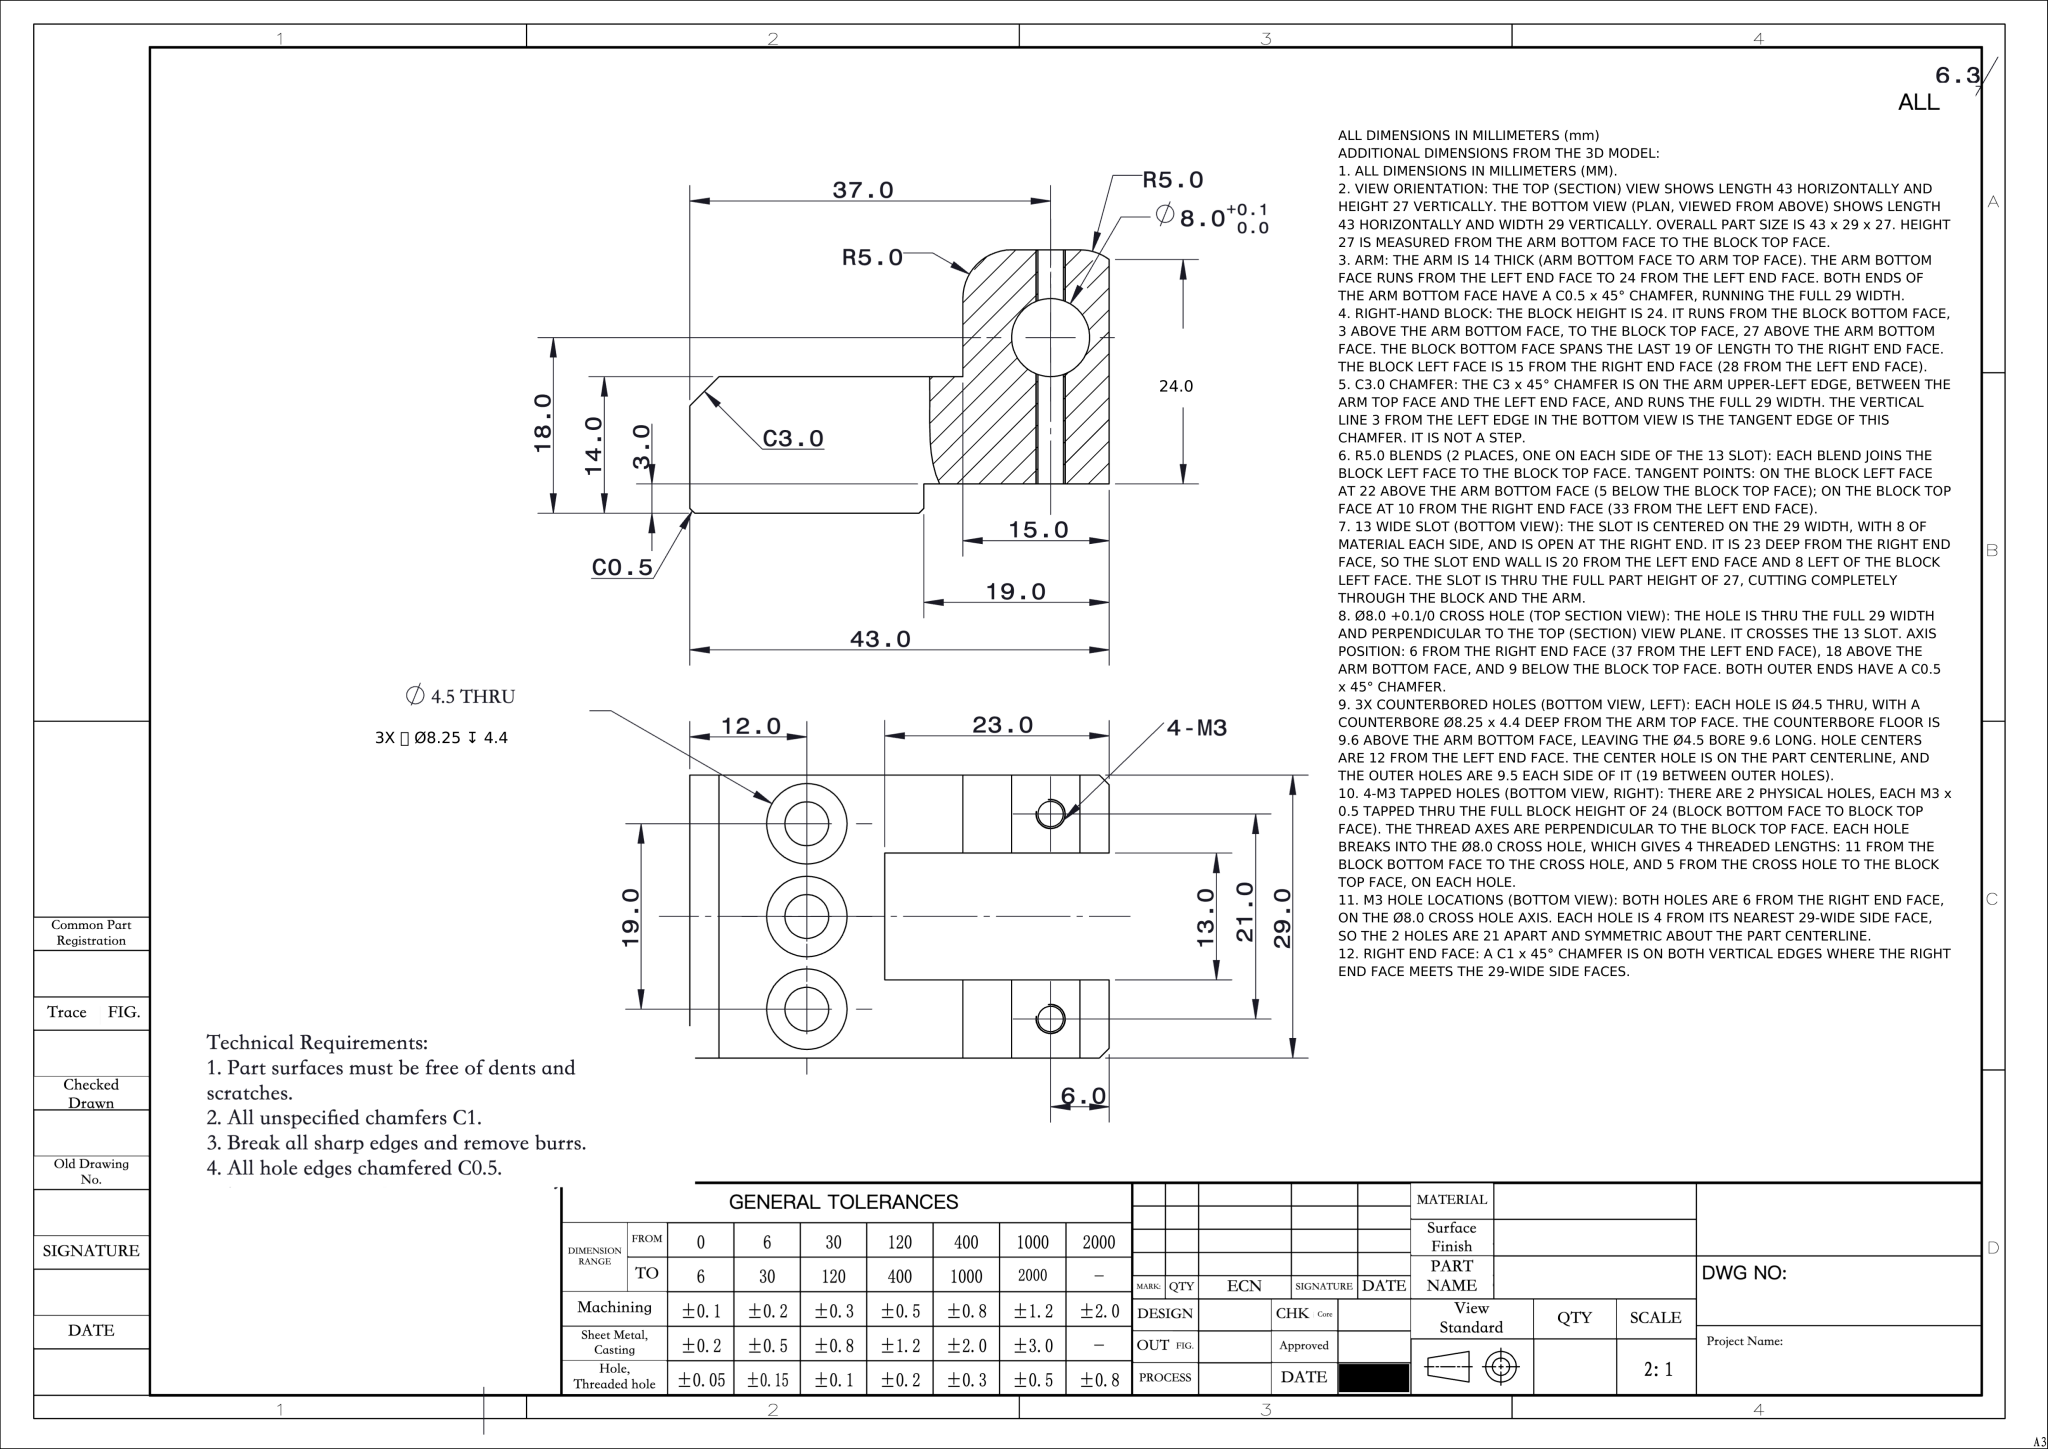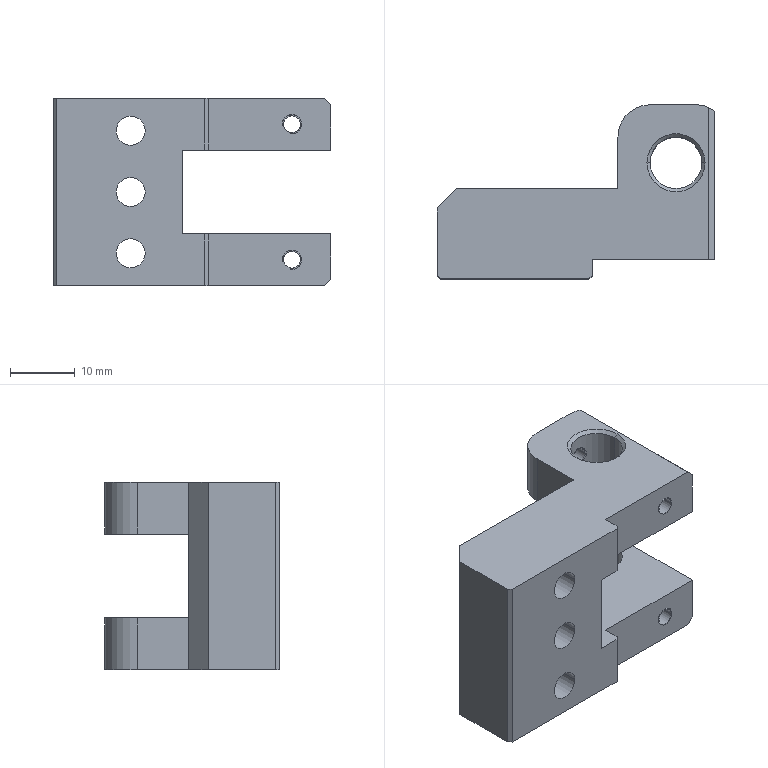Part | NX | mm | 1 solid | 91 faces | box 43 x 27 x 29 mm | volume 13068 mm3 | cylinder 52 | plane 35 | cone 4 | commonest cylinder face diameters 2.949 x12 3 x12 2.6 x8 4.5 x6 8.25 x6 8 x4 10 x4